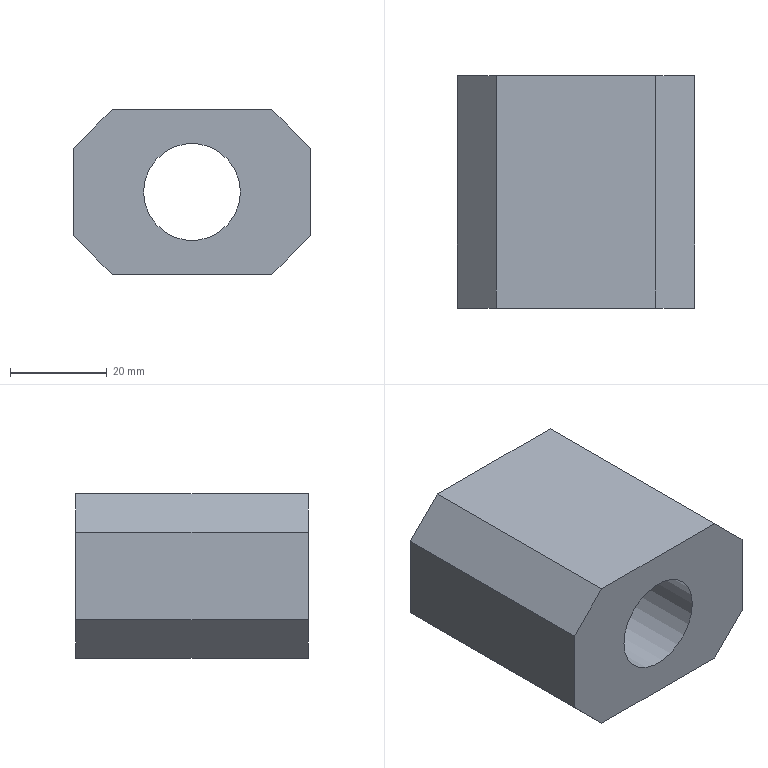Component | NX | NUT | 1 solid | 11 faces | box 49 x 48 x 34 mm | volume 58744 mm3 | plane 10 | cylinder 1 | commonest cylinder face diameters 20 x1
STEP:
#1=CARTESIAN_POINT('',(0.,0.,0.));
#2=DIRECTION('',(0.,0.,1.));
#3=DIRECTION('',(1.,0.,0.));
#4=AXIS2_PLACEMENT_3D('',#1,#2,#3);
#5=CARTESIAN_POINT('',(29.335,31.63,45.));
#6=VERTEX_POINT('',#5);
#7=CARTESIAN_POINT('',(29.335,31.63,63.));
#8=VERTEX_POINT('',#7);
#9=CARTESIAN_POINT('',(29.335,31.63,37.));
#10=DIRECTION('',(0.,0.,1.));
#11=VECTOR('',#10,1.);
#12=LINE('',#9,#11);
#13=CARTESIAN_POINT('',(29.335,-16.37,37.));
#14=DIRECTION('',(-1.,0.,0.));
#15=DIRECTION('',(0.,-1.,0.));
#16=AXIS2_PLACEMENT_3D('',#13,#14,#15);
#17=PLANE('',#16);
#18=CARTESIAN_POINT('',(-48.,0.));
#19=DIRECTION('',(0.,1.));
#20=VECTOR('',#19,1.);
#21=LINE('',#18,#20);
#22=(GEOMETRIC_REPRESENTATION_CONTEXT(2)PARAMETRIC_REPRESENTATION_CONTEXT()REPRESENTATION_CONTEXT('',''));
#23=DEFINITIONAL_REPRESENTATION('',(#21),#22);
#24=PCURVE('',#17,#23);
#25=CARTESIAN_POINT('',(4.835,31.63,54.));
#26=DIRECTION('',(0.,-1.,0.));
#27=DIRECTION('',(1.,0.,0.));
#28=AXIS2_PLACEMENT_3D('',#25,#26,#27);
#29=PLANE('',#28);
#30=CARTESIAN_POINT('',(24.5,-17.));
#31=DIRECTION('',(0.,1.));
#32=VECTOR('',#31,1.);
#33=LINE('',#30,#32);
#34=(GEOMETRIC_REPRESENTATION_CONTEXT(2)PARAMETRIC_REPRESENTATION_CONTEXT()REPRESENTATION_CONTEXT('',''));
#35=DEFINITIONAL_REPRESENTATION('',(#33),#34);
#36=PCURVE('',#29,#35);
#37=SURFACE_CURVE('',#12,(#24,#36),.PCURVE_S1.);
#38=EDGE_CURVE('',#6,#8,#37,.T.);
#39=ORIENTED_EDGE('',*,*,#38,.T.);
#40=CARTESIAN_POINT('',(29.335,-16.37,63.));
#41=VERTEX_POINT('',#40);
#42=CARTESIAN_POINT('',(29.335,-16.37,63.));
#43=DIRECTION('',(0.,-1.,0.));
#44=VECTOR('',#43,1.);
#45=LINE('',#42,#44);
#46=CARTESIAN_POINT('',(0.,26.));
#47=DIRECTION('',(1.,0.));
#48=VECTOR('',#47,1.);
#49=LINE('',#46,#48);
#50=(GEOMETRIC_REPRESENTATION_CONTEXT(2)PARAMETRIC_REPRESENTATION_CONTEXT()REPRESENTATION_CONTEXT('',''));
#51=DEFINITIONAL_REPRESENTATION('',(#49),#50);
#52=PCURVE('',#17,#51);
#53=CARTESIAN_POINT('',(21.335,-16.37,71.));
#54=DIRECTION('',(-0.7071,0.,-0.7071));
#55=DIRECTION('',(0.,1.,0.));
#56=AXIS2_PLACEMENT_3D('',#53,#54,#55);
#57=PLANE('',#56);
#58=CARTESIAN_POINT('',(0.,11.314));
#59=DIRECTION('',(-1.,0.));
#60=VECTOR('',#59,1.);
#61=LINE('',#58,#60);
#62=(GEOMETRIC_REPRESENTATION_CONTEXT(2)PARAMETRIC_REPRESENTATION_CONTEXT()REPRESENTATION_CONTEXT('',''));
#63=DEFINITIONAL_REPRESENTATION('',(#61),#62);
#64=PCURVE('',#57,#63);
#65=SURFACE_CURVE('',#45,(#52,#64),.PCURVE_S1.);
#66=EDGE_CURVE('',#8,#41,#65,.T.);
#67=ORIENTED_EDGE('',*,*,#66,.T.);
#68=CARTESIAN_POINT('',(29.335,-16.37,45.));
#69=VERTEX_POINT('',#68);
#70=CARTESIAN_POINT('',(29.335,-16.37,37.));
#71=DIRECTION('',(0.,0.,1.));
#72=VECTOR('',#71,1.);
#73=LINE('',#70,#72);
#74=CARTESIAN_POINT('',(0.,0.));
#75=DIRECTION('',(0.,1.));
#76=VECTOR('',#75,1.);
#77=LINE('',#74,#76);
#78=(GEOMETRIC_REPRESENTATION_CONTEXT(2)PARAMETRIC_REPRESENTATION_CONTEXT()REPRESENTATION_CONTEXT('',''));
#79=DEFINITIONAL_REPRESENTATION('',(#77),#78);
#80=PCURVE('',#17,#79);
#81=CARTESIAN_POINT('',(4.835,-16.37,54.));
#82=DIRECTION('',(0.,-1.,0.));
#83=DIRECTION('',(1.,0.,0.));
#84=AXIS2_PLACEMENT_3D('',#81,#82,#83);
#85=PLANE('',#84);
#86=CARTESIAN_POINT('',(24.5,-17.));
#87=DIRECTION('',(0.,1.));
#88=VECTOR('',#87,1.);
#89=LINE('',#86,#88);
#90=(GEOMETRIC_REPRESENTATION_CONTEXT(2)PARAMETRIC_REPRESENTATION_CONTEXT()REPRESENTATION_CONTEXT('',''));
#91=DEFINITIONAL_REPRESENTATION('',(#89),#90);
#92=PCURVE('',#85,#91);
#93=SURFACE_CURVE('',#73,(#80,#92),.PCURVE_S1.);
#94=EDGE_CURVE('',#69,#41,#93,.T.);
#95=ORIENTED_EDGE('',*,*,#94,.F.);
#96=CARTESIAN_POINT('',(29.335,-16.37,45.));
#97=DIRECTION('',(0.,1.,0.));
#98=VECTOR('',#97,1.);
#99=LINE('',#96,#98);
#100=CARTESIAN_POINT('',(0.,8.));
#101=DIRECTION('',(-1.,0.));
#102=VECTOR('',#101,1.);
#103=LINE('',#100,#102);
#104=(GEOMETRIC_REPRESENTATION_CONTEXT(2)PARAMETRIC_REPRESENTATION_CONTEXT()REPRESENTATION_CONTEXT('',''));
#105=DEFINITIONAL_REPRESENTATION('',(#103),#104);
#106=PCURVE('',#17,#105);
#107=CARTESIAN_POINT('',(29.335,-16.37,45.));
#108=DIRECTION('',(-0.7071,0.,0.7071));
#109=DIRECTION('',(0.,1.,0.));
#110=AXIS2_PLACEMENT_3D('',#107,#108,#109);
#111=PLANE('',#110);
#112=CARTESIAN_POINT('',(0.,0.));
#113=DIRECTION('',(1.,0.));
#114=VECTOR('',#113,1.);
#115=LINE('',#112,#114);
#116=(GEOMETRIC_REPRESENTATION_CONTEXT(2)PARAMETRIC_REPRESENTATION_CONTEXT()REPRESENTATION_CONTEXT('',''));
#117=DEFINITIONAL_REPRESENTATION('',(#115),#116);
#118=PCURVE('',#111,#117);
#119=SURFACE_CURVE('',#99,(#106,#118),.PCURVE_S1.);
#120=EDGE_CURVE('',#69,#6,#119,.T.);
#121=ORIENTED_EDGE('',*,*,#120,.T.);
#122=EDGE_LOOP('',(#39,#67,#95,#121));
#123=FACE_BOUND('',#122,.T.);
#124=ADVANCED_FACE('',(#123),#17,.F.);
#125=CARTESIAN_POINT('',(21.335,31.63,71.));
#126=VERTEX_POINT('',#125);
#127=CARTESIAN_POINT('',(-11.665,31.63,71.));
#128=VERTEX_POINT('',#127);
#129=CARTESIAN_POINT('',(29.335,31.63,71.));
#130=DIRECTION('',(-1.,0.,0.));
#131=VECTOR('',#130,1.);
#132=LINE('',#129,#131);
#133=CARTESIAN_POINT('',(29.335,-16.37,71.));
#134=DIRECTION('',(0.,0.,-1.));
#135=DIRECTION('',(0.,1.,0.));
#136=AXIS2_PLACEMENT_3D('',#133,#134,#135);
#137=PLANE('',#136);
#138=CARTESIAN_POINT('',(48.,0.));
#139=DIRECTION('',(0.,-1.));
#140=VECTOR('',#139,1.);
#141=LINE('',#138,#140);
#142=(GEOMETRIC_REPRESENTATION_CONTEXT(2)PARAMETRIC_REPRESENTATION_CONTEXT()REPRESENTATION_CONTEXT('',''));
#143=DEFINITIONAL_REPRESENTATION('',(#141),#142);
#144=PCURVE('',#137,#143);
#145=CARTESIAN_POINT('',(24.5,17.));
#146=DIRECTION('',(-1.,0.));
#147=VECTOR('',#146,1.);
#148=LINE('',#145,#147);
#149=(GEOMETRIC_REPRESENTATION_CONTEXT(2)PARAMETRIC_REPRESENTATION_CONTEXT()REPRESENTATION_CONTEXT('',''));
#150=DEFINITIONAL_REPRESENTATION('',(#148),#149);
#151=PCURVE('',#29,#150);
#152=SURFACE_CURVE('',#132,(#144,#151),.PCURVE_S1.);
#153=EDGE_CURVE('',#126,#128,#152,.T.);
#154=ORIENTED_EDGE('',*,*,#153,.T.);
#155=CARTESIAN_POINT('',(-11.665,-16.37,71.));
#156=VERTEX_POINT('',#155);
#157=CARTESIAN_POINT('',(-11.665,-16.37,71.));
#158=DIRECTION('',(0.,-1.,0.));
#159=VECTOR('',#158,1.);
#160=LINE('',#157,#159);
#161=CARTESIAN_POINT('',(0.,-41.));
#162=DIRECTION('',(-1.,0.));
#163=VECTOR('',#162,1.);
#164=LINE('',#161,#163);
#165=(GEOMETRIC_REPRESENTATION_CONTEXT(2)PARAMETRIC_REPRESENTATION_CONTEXT()REPRESENTATION_CONTEXT('',''));
#166=DEFINITIONAL_REPRESENTATION('',(#164),#165);
#167=PCURVE('',#137,#166);
#168=CARTESIAN_POINT('',(-19.665,-16.37,63.));
#169=DIRECTION('',(0.7071,0.,-0.7071));
#170=DIRECTION('',(0.,1.,0.));
#171=AXIS2_PLACEMENT_3D('',#168,#169,#170);
#172=PLANE('',#171);
#173=CARTESIAN_POINT('',(0.,11.314));
#174=DIRECTION('',(-1.,0.));
#175=VECTOR('',#174,1.);
#176=LINE('',#173,#175);
#177=(GEOMETRIC_REPRESENTATION_CONTEXT(2)PARAMETRIC_REPRESENTATION_CONTEXT()REPRESENTATION_CONTEXT('',''));
#178=DEFINITIONAL_REPRESENTATION('',(#176),#177);
#179=PCURVE('',#172,#178);
#180=SURFACE_CURVE('',#160,(#167,#179),.PCURVE_S1.);
#181=EDGE_CURVE('',#128,#156,#180,.T.);
#182=ORIENTED_EDGE('',*,*,#181,.T.);
#183=CARTESIAN_POINT('',(21.335,-16.37,71.));
#184=VERTEX_POINT('',#183);
#185=CARTESIAN_POINT('',(29.335,-16.37,71.));
#186=DIRECTION('',(-1.,0.,0.));
#187=VECTOR('',#186,1.);
#188=LINE('',#185,#187);
#189=CARTESIAN_POINT('',(0.,0.));
#190=DIRECTION('',(0.,-1.));
#191=VECTOR('',#190,1.);
#192=LINE('',#189,#191);
#193=(GEOMETRIC_REPRESENTATION_CONTEXT(2)PARAMETRIC_REPRESENTATION_CONTEXT()REPRESENTATION_CONTEXT('',''));
#194=DEFINITIONAL_REPRESENTATION('',(#192),#193);
#195=PCURVE('',#137,#194);
#196=CARTESIAN_POINT('',(24.5,17.));
#197=DIRECTION('',(-1.,0.));
#198=VECTOR('',#197,1.);
#199=LINE('',#196,#198);
#200=(GEOMETRIC_REPRESENTATION_CONTEXT(2)PARAMETRIC_REPRESENTATION_CONTEXT()REPRESENTATION_CONTEXT('',''));
#201=DEFINITIONAL_REPRESENTATION('',(#199),#200);
#202=PCURVE('',#85,#201);
#203=SURFACE_CURVE('',#188,(#195,#202),.PCURVE_S1.);
#204=EDGE_CURVE('',#184,#156,#203,.T.);
#205=ORIENTED_EDGE('',*,*,#204,.F.);
#206=CARTESIAN_POINT('',(21.335,-16.37,71.));
#207=DIRECTION('',(0.,1.,0.));
#208=VECTOR('',#207,1.);
#209=LINE('',#206,#208);
#210=CARTESIAN_POINT('',(0.,-8.));
#211=DIRECTION('',(1.,0.));
#212=VECTOR('',#211,1.);
#213=LINE('',#210,#212);
#214=(GEOMETRIC_REPRESENTATION_CONTEXT(2)PARAMETRIC_REPRESENTATION_CONTEXT()REPRESENTATION_CONTEXT('',''));
#215=DEFINITIONAL_REPRESENTATION('',(#213),#214);
#216=PCURVE('',#137,#215);
#217=CARTESIAN_POINT('',(0.,0.));
#218=DIRECTION('',(1.,0.));
#219=VECTOR('',#218,1.);
#220=LINE('',#217,#219);
#221=(GEOMETRIC_REPRESENTATION_CONTEXT(2)PARAMETRIC_REPRESENTATION_CONTEXT()REPRESENTATION_CONTEXT('',''));
#222=DEFINITIONAL_REPRESENTATION('',(#220),#221);
#223=PCURVE('',#57,#222);
#224=SURFACE_CURVE('',#209,(#216,#223),.PCURVE_S1.);
#225=EDGE_CURVE('',#184,#126,#224,.T.);
#226=ORIENTED_EDGE('',*,*,#225,.T.);
#227=EDGE_LOOP('',(#154,#182,#205,#226));
#228=FACE_BOUND('',#227,.T.);
#229=ADVANCED_FACE('',(#228),#137,.F.);
#230=CARTESIAN_POINT('',(-19.665,-16.37,63.));
#231=VERTEX_POINT('',#230);
#232=CARTESIAN_POINT('',(-19.665,-16.37,45.));
#233=VERTEX_POINT('',#232);
#234=CARTESIAN_POINT('',(-19.665,-16.37,71.));
#235=DIRECTION('',(0.,0.,-1.));
#236=VECTOR('',#235,1.);
#237=LINE('',#234,#236);
#238=CARTESIAN_POINT('',(-19.665,-16.37,71.));
#239=DIRECTION('',(1.,0.,0.));
#240=DIRECTION('',(0.,1.,0.));
#241=AXIS2_PLACEMENT_3D('',#238,#239,#240);
#242=PLANE('',#241);
#243=CARTESIAN_POINT('',(0.,0.));
#244=DIRECTION('',(0.,-1.));
#245=VECTOR('',#244,1.);
#246=LINE('',#243,#245);
#247=(GEOMETRIC_REPRESENTATION_CONTEXT(2)PARAMETRIC_REPRESENTATION_CONTEXT()REPRESENTATION_CONTEXT('',''));
#248=DEFINITIONAL_REPRESENTATION('',(#246),#247);
#249=PCURVE('',#242,#248);
#250=CARTESIAN_POINT('',(-24.5,17.));
#251=DIRECTION('',(0.,-1.));
#252=VECTOR('',#251,1.);
#253=LINE('',#250,#252);
#254=(GEOMETRIC_REPRESENTATION_CONTEXT(2)PARAMETRIC_REPRESENTATION_CONTEXT()REPRESENTATION_CONTEXT('',''));
#255=DEFINITIONAL_REPRESENTATION('',(#253),#254);
#256=PCURVE('',#85,#255);
#257=SURFACE_CURVE('',#237,(#249,#256),.PCURVE_S1.);
#258=EDGE_CURVE('',#231,#233,#257,.T.);
#259=ORIENTED_EDGE('',*,*,#258,.F.);
#260=CARTESIAN_POINT('',(-19.665,31.63,63.));
#261=VERTEX_POINT('',#260);
#262=CARTESIAN_POINT('',(-19.665,-16.37,63.));
#263=DIRECTION('',(0.,1.,0.));
#264=VECTOR('',#263,1.);
#265=LINE('',#262,#264);
#266=CARTESIAN_POINT('',(0.,-8.));
#267=DIRECTION('',(1.,0.));
#268=VECTOR('',#267,1.);
#269=LINE('',#266,#268);
#270=(GEOMETRIC_REPRESENTATION_CONTEXT(2)PARAMETRIC_REPRESENTATION_CONTEXT()REPRESENTATION_CONTEXT('',''));
#271=DEFINITIONAL_REPRESENTATION('',(#269),#270);
#272=PCURVE('',#242,#271);
#273=CARTESIAN_POINT('',(0.,0.));
#274=DIRECTION('',(1.,0.));
#275=VECTOR('',#274,1.);
#276=LINE('',#273,#275);
#277=(GEOMETRIC_REPRESENTATION_CONTEXT(2)PARAMETRIC_REPRESENTATION_CONTEXT()REPRESENTATION_CONTEXT('',''));
#278=DEFINITIONAL_REPRESENTATION('',(#276),#277);
#279=PCURVE('',#172,#278);
#280=SURFACE_CURVE('',#265,(#272,#279),.PCURVE_S1.);
#281=EDGE_CURVE('',#231,#261,#280,.T.);
#282=ORIENTED_EDGE('',*,*,#281,.T.);
#283=CARTESIAN_POINT('',(-19.665,31.63,45.));
#284=VERTEX_POINT('',#283);
#285=CARTESIAN_POINT('',(-19.665,31.63,71.));
#286=DIRECTION('',(0.,0.,-1.));
#287=VECTOR('',#286,1.);
#288=LINE('',#285,#287);
#289=CARTESIAN_POINT('',(48.,0.));
#290=DIRECTION('',(0.,-1.));
#291=VECTOR('',#290,1.);
#292=LINE('',#289,#291);
#293=(GEOMETRIC_REPRESENTATION_CONTEXT(2)PARAMETRIC_REPRESENTATION_CONTEXT()REPRESENTATION_CONTEXT('',''));
#294=DEFINITIONAL_REPRESENTATION('',(#292),#293);
#295=PCURVE('',#242,#294);
#296=CARTESIAN_POINT('',(-24.5,17.));
#297=DIRECTION('',(0.,-1.));
#298=VECTOR('',#297,1.);
#299=LINE('',#296,#298);
#300=(GEOMETRIC_REPRESENTATION_CONTEXT(2)PARAMETRIC_REPRESENTATION_CONTEXT()REPRESENTATION_CONTEXT('',''));
#301=DEFINITIONAL_REPRESENTATION('',(#299),#300);
#302=PCURVE('',#29,#301);
#303=SURFACE_CURVE('',#288,(#295,#302),.PCURVE_S1.);
#304=EDGE_CURVE('',#261,#284,#303,.T.);
#305=ORIENTED_EDGE('',*,*,#304,.T.);
#306=CARTESIAN_POINT('',(-19.665,-16.37,45.));
#307=DIRECTION('',(0.,-1.,0.));
#308=VECTOR('',#307,1.);
#309=LINE('',#306,#308);
#310=CARTESIAN_POINT('',(0.,-26.));
#311=DIRECTION('',(-1.,0.));
#312=VECTOR('',#311,1.);
#313=LINE('',#310,#312);
#314=(GEOMETRIC_REPRESENTATION_CONTEXT(2)PARAMETRIC_REPRESENTATION_CONTEXT()REPRESENTATION_CONTEXT('',''));
#315=DEFINITIONAL_REPRESENTATION('',(#313),#314);
#316=PCURVE('',#242,#315);
#317=CARTESIAN_POINT('',(-11.665,-16.37,37.));
#318=DIRECTION('',(0.7071,0.,0.7071));
#319=DIRECTION('',(0.,1.,0.));
#320=AXIS2_PLACEMENT_3D('',#317,#318,#319);
#321=PLANE('',#320);
#322=CARTESIAN_POINT('',(0.,11.314));
#323=DIRECTION('',(-1.,0.));
#324=VECTOR('',#323,1.);
#325=LINE('',#322,#324);
#326=(GEOMETRIC_REPRESENTATION_CONTEXT(2)PARAMETRIC_REPRESENTATION_CONTEXT()REPRESENTATION_CONTEXT('',''));
#327=DEFINITIONAL_REPRESENTATION('',(#325),#326);
#328=PCURVE('',#321,#327);
#329=SURFACE_CURVE('',#309,(#316,#328),.PCURVE_S1.);
#330=EDGE_CURVE('',#284,#233,#329,.T.);
#331=ORIENTED_EDGE('',*,*,#330,.T.);
#332=EDGE_LOOP('',(#259,#282,#305,#331));
#333=FACE_BOUND('',#332,.T.);
#334=ADVANCED_FACE('',(#333),#242,.F.);
#335=CARTESIAN_POINT('',(-11.665,-16.37,37.));
#336=VERTEX_POINT('',#335);
#337=CARTESIAN_POINT('',(21.335,-16.37,37.));
#338=VERTEX_POINT('',#337);
#339=CARTESIAN_POINT('',(-19.665,-16.37,37.));
#340=DIRECTION('',(1.,0.,0.));
#341=VECTOR('',#340,1.);
#342=LINE('',#339,#341);
#343=CARTESIAN_POINT('',(-19.665,-16.37,37.));
#344=DIRECTION('',(0.,0.,1.));
#345=DIRECTION('',(0.,-1.,0.));
#346=AXIS2_PLACEMENT_3D('',#343,#344,#345);
#347=PLANE('',#346);
#348=CARTESIAN_POINT('',(0.,0.));
#349=DIRECTION('',(0.,1.));
#350=VECTOR('',#349,1.);
#351=LINE('',#348,#350);
#352=(GEOMETRIC_REPRESENTATION_CONTEXT(2)PARAMETRIC_REPRESENTATION_CONTEXT()REPRESENTATION_CONTEXT('',''));
#353=DEFINITIONAL_REPRESENTATION('',(#351),#352);
#354=PCURVE('',#347,#353);
#355=CARTESIAN_POINT('',(-24.5,-17.));
#356=DIRECTION('',(1.,0.));
#357=VECTOR('',#356,1.);
#358=LINE('',#355,#357);
#359=(GEOMETRIC_REPRESENTATION_CONTEXT(2)PARAMETRIC_REPRESENTATION_CONTEXT()REPRESENTATION_CONTEXT('',''));
#360=DEFINITIONAL_REPRESENTATION('',(#358),#359);
#361=PCURVE('',#85,#360);
#362=SURFACE_CURVE('',#342,(#354,#361),.PCURVE_S1.);
#363=EDGE_CURVE('',#336,#338,#362,.T.);
#364=ORIENTED_EDGE('',*,*,#363,.F.);
#365=CARTESIAN_POINT('',(-11.665,31.63,37.));
#366=VERTEX_POINT('',#365);
#367=CARTESIAN_POINT('',(-11.665,-16.37,37.));
#368=DIRECTION('',(0.,1.,0.));
#369=VECTOR('',#368,1.);
#370=LINE('',#367,#369);
#371=CARTESIAN_POINT('',(0.,8.));
#372=DIRECTION('',(-1.,0.));
#373=VECTOR('',#372,1.);
#374=LINE('',#371,#373);
#375=(GEOMETRIC_REPRESENTATION_CONTEXT(2)PARAMETRIC_REPRESENTATION_CONTEXT()REPRESENTATION_CONTEXT('',''));
#376=DEFINITIONAL_REPRESENTATION('',(#374),#375);
#377=PCURVE('',#347,#376);
#378=CARTESIAN_POINT('',(0.,0.));
#379=DIRECTION('',(1.,0.));
#380=VECTOR('',#379,1.);
#381=LINE('',#378,#380);
#382=(GEOMETRIC_REPRESENTATION_CONTEXT(2)PARAMETRIC_REPRESENTATION_CONTEXT()REPRESENTATION_CONTEXT('',''));
#383=DEFINITIONAL_REPRESENTATION('',(#381),#382);
#384=PCURVE('',#321,#383);
#385=SURFACE_CURVE('',#370,(#377,#384),.PCURVE_S1.);
#386=EDGE_CURVE('',#336,#366,#385,.T.);
#387=ORIENTED_EDGE('',*,*,#386,.T.);
#388=CARTESIAN_POINT('',(21.335,31.63,37.));
#389=VERTEX_POINT('',#388);
#390=CARTESIAN_POINT('',(-19.665,31.63,37.));
#391=DIRECTION('',(1.,0.,0.));
#392=VECTOR('',#391,1.);
#393=LINE('',#390,#392);
#394=CARTESIAN_POINT('',(-48.,0.));
#395=DIRECTION('',(0.,1.));
#396=VECTOR('',#395,1.);
#397=LINE('',#394,#396);
#398=(GEOMETRIC_REPRESENTATION_CONTEXT(2)PARAMETRIC_REPRESENTATION_CONTEXT()REPRESENTATION_CONTEXT('',''));
#399=DEFINITIONAL_REPRESENTATION('',(#397),#398);
#400=PCURVE('',#347,#399);
#401=CARTESIAN_POINT('',(-24.5,-17.));
#402=DIRECTION('',(1.,0.));
#403=VECTOR('',#402,1.);
#404=LINE('',#401,#403);
#405=(GEOMETRIC_REPRESENTATION_CONTEXT(2)PARAMETRIC_REPRESENTATION_CONTEXT()REPRESENTATION_CONTEXT('',''));
#406=DEFINITIONAL_REPRESENTATION('',(#404),#405);
#407=PCURVE('',#29,#406);
#408=SURFACE_CURVE('',#393,(#400,#407),.PCURVE_S1.);
#409=EDGE_CURVE('',#366,#389,#408,.T.);
#410=ORIENTED_EDGE('',*,*,#409,.T.);
#411=CARTESIAN_POINT('',(21.335,-16.37,37.));
#412=DIRECTION('',(0.,-1.,0.));
#413=VECTOR('',#412,1.);
#414=LINE('',#411,#413);
#415=CARTESIAN_POINT('',(0.,41.));
#416=DIRECTION('',(1.,0.));
#417=VECTOR('',#416,1.);
#418=LINE('',#415,#417);
#419=(GEOMETRIC_REPRESENTATION_CONTEXT(2)PARAMETRIC_REPRESENTATION_CONTEXT()REPRESENTATION_CONTEXT('',''));
#420=DEFINITIONAL_REPRESENTATION('',(#418),#419);
#421=PCURVE('',#347,#420);
#422=CARTESIAN_POINT('',(0.,11.314));
#423=DIRECTION('',(-1.,0.));
#424=VECTOR('',#423,1.);
#425=LINE('',#422,#424);
#426=(GEOMETRIC_REPRESENTATION_CONTEXT(2)PARAMETRIC_REPRESENTATION_CONTEXT()REPRESENTATION_CONTEXT('',''));
#427=DEFINITIONAL_REPRESENTATION('',(#425),#426);
#428=PCURVE('',#111,#427);
#429=SURFACE_CURVE('',#414,(#421,#428),.PCURVE_S1.);
#430=EDGE_CURVE('',#389,#338,#429,.T.);
#431=ORIENTED_EDGE('',*,*,#430,.T.);
#432=EDGE_LOOP('',(#364,#387,#410,#431));
#433=FACE_BOUND('',#432,.T.);
#434=ADVANCED_FACE('',(#433),#347,.F.);
#435=CARTESIAN_POINT('',(14.835,-16.37,54.));
#436=VERTEX_POINT('',#435);
#437=CARTESIAN_POINT('',(4.835,-16.37,54.));
#438=DIRECTION('',(0.,-1.,0.));
#439=DIRECTION('',(1.,0.,0.));
#440=AXIS2_PLACEMENT_3D('',#437,#438,#439);
#441=CIRCLE('',#440,10.);
#442=CARTESIAN_POINT('',(0.,0.));
#443=DIRECTION('',(1.,0.));
#444=AXIS2_PLACEMENT_2D('',#442,#443);
#445=CIRCLE('',#444,10.);
#446=(GEOMETRIC_REPRESENTATION_CONTEXT(2)PARAMETRIC_REPRESENTATION_CONTEXT()REPRESENTATION_CONTEXT('',''));
#447=DEFINITIONAL_REPRESENTATION('',(#445),#446);
#448=PCURVE('',#85,#447);
#449=CARTESIAN_POINT('',(4.835,31.63,54.));
#450=DIRECTION('',(0.,-1.,0.));
#451=DIRECTION('',(1.,0.,0.));
#452=AXIS2_PLACEMENT_3D('',#449,#450,#451);
#453=CYLINDRICAL_SURFACE('',#452,10.);
#454=CARTESIAN_POINT('',(0.,48.));
#455=DIRECTION('',(1.,0.));
#456=VECTOR('',#455,1.);
#457=LINE('',#454,#456);
#458=(GEOMETRIC_REPRESENTATION_CONTEXT(2)PARAMETRIC_REPRESENTATION_CONTEXT()REPRESENTATION_CONTEXT('',''));
#459=DEFINITIONAL_REPRESENTATION('',(#457),#458);
#460=PCURVE('',#453,#459);
#461=SURFACE_CURVE('',#441,(#448,#460),.PCURVE_S1.);
#462=EDGE_CURVE('',#436,#436,#461,.T.);
#463=ORIENTED_EDGE('',*,*,#462,.F.);
#464=EDGE_LOOP('',(#463));
#465=FACE_BOUND('',#464,.T.);
#466=ORIENTED_EDGE('',*,*,#204,.T.);
#467=CARTESIAN_POINT('',(-11.915,-16.37,70.75));
#468=DIRECTION('',(-0.7071,0.,-0.7071));
#469=VECTOR('',#468,1.);
#470=LINE('',#467,#469);
#471=CARTESIAN_POINT('',(-16.75,16.75));
#472=DIRECTION('',(-0.7071,-0.7071));
#473=VECTOR('',#472,1.);
#474=LINE('',#471,#473);
#475=(GEOMETRIC_REPRESENTATION_CONTEXT(2)PARAMETRIC_REPRESENTATION_CONTEXT()REPRESENTATION_CONTEXT('',''));
#476=DEFINITIONAL_REPRESENTATION('',(#474),#475);
#477=PCURVE('',#85,#476);
#478=CARTESIAN_POINT('',(0.,10.96));
#479=DIRECTION('',(0.,-1.));
#480=VECTOR('',#479,1.);
#481=LINE('',#478,#480);
#482=(GEOMETRIC_REPRESENTATION_CONTEXT(2)PARAMETRIC_REPRESENTATION_CONTEXT()REPRESENTATION_CONTEXT('',''));
#483=DEFINITIONAL_REPRESENTATION('',(#481),#482);
#484=PCURVE('',#172,#483);
#485=SURFACE_CURVE('',#470,(#477,#484),.PCURVE_S1.);
#486=EDGE_CURVE('',#156,#231,#485,.T.);
#487=ORIENTED_EDGE('',*,*,#486,.T.);
#488=ORIENTED_EDGE('',*,*,#258,.T.);
#489=CARTESIAN_POINT('',(-11.915,-16.37,37.25));
#490=DIRECTION('',(0.7071,0.,-0.7071));
#491=VECTOR('',#490,1.);
#492=LINE('',#489,#491);
#493=CARTESIAN_POINT('',(-16.75,-16.75));
#494=DIRECTION('',(0.7071,-0.7071));
#495=VECTOR('',#494,1.);
#496=LINE('',#493,#495);
#497=(GEOMETRIC_REPRESENTATION_CONTEXT(2)PARAMETRIC_REPRESENTATION_CONTEXT()REPRESENTATION_CONTEXT('',''));
#498=DEFINITIONAL_REPRESENTATION('',(#496),#497);
#499=PCURVE('',#85,#498);
#500=CARTESIAN_POINT('',(0.,0.3536));
#501=DIRECTION('',(0.,-1.));
#502=VECTOR('',#501,1.);
#503=LINE('',#500,#502);
#504=(GEOMETRIC_REPRESENTATION_CONTEXT(2)PARAMETRIC_REPRESENTATION_CONTEXT()REPRESENTATION_CONTEXT('',''));
#505=DEFINITIONAL_REPRESENTATION('',(#503),#504);
#506=PCURVE('',#321,#505);
#507=SURFACE_CURVE('',#492,(#499,#506),.PCURVE_S1.);
#508=EDGE_CURVE('',#233,#336,#507,.T.);
#509=ORIENTED_EDGE('',*,*,#508,.T.);
#510=ORIENTED_EDGE('',*,*,#363,.T.);
#511=CARTESIAN_POINT('',(21.585,-16.37,37.25));
#512=DIRECTION('',(0.7071,0.,0.7071));
#513=VECTOR('',#512,1.);
#514=LINE('',#511,#513);
#515=CARTESIAN_POINT('',(16.75,-16.75));
#516=DIRECTION('',(0.7071,0.7071));
#517=VECTOR('',#516,1.);
#518=LINE('',#515,#517);
#519=(GEOMETRIC_REPRESENTATION_CONTEXT(2)PARAMETRIC_REPRESENTATION_CONTEXT()REPRESENTATION_CONTEXT('',''));
#520=DEFINITIONAL_REPRESENTATION('',(#518),#519);
#521=PCURVE('',#85,#520);
#522=CARTESIAN_POINT('',(0.,10.96));
#523=DIRECTION('',(0.,-1.));
#524=VECTOR('',#523,1.);
#525=LINE('',#522,#524);
#526=(GEOMETRIC_REPRESENTATION_CONTEXT(2)PARAMETRIC_REPRESENTATION_CONTEXT()REPRESENTATION_CONTEXT('',''));
#527=DEFINITIONAL_REPRESENTATION('',(#525),#526);
#528=PCURVE('',#111,#527);
#529=SURFACE_CURVE('',#514,(#521,#528),.PCURVE_S1.);
#530=EDGE_CURVE('',#338,#69,#529,.T.);
#531=ORIENTED_EDGE('',*,*,#530,.T.);
#532=ORIENTED_EDGE('',*,*,#94,.T.);
#533=CARTESIAN_POINT('',(21.585,-16.37,70.75));
#534=DIRECTION('',(-0.7071,0.,0.7071));
#535=VECTOR('',#534,1.);
#536=LINE('',#533,#535);
#537=CARTESIAN_POINT('',(16.75,16.75));
#538=DIRECTION('',(-0.7071,0.7071));
#539=VECTOR('',#538,1.);
#540=LINE('',#537,#539);
#541=(GEOMETRIC_REPRESENTATION_CONTEXT(2)PARAMETRIC_REPRESENTATION_CONTEXT()REPRESENTATION_CONTEXT('',''));
#542=DEFINITIONAL_REPRESENTATION('',(#540),#541);
#543=PCURVE('',#85,#542);
#544=CARTESIAN_POINT('',(0.,0.3536));
#545=DIRECTION('',(0.,-1.));
#546=VECTOR('',#545,1.);
#547=LINE('',#544,#546);
#548=(GEOMETRIC_REPRESENTATION_CONTEXT(2)PARAMETRIC_REPRESENTATION_CONTEXT()REPRESENTATION_CONTEXT('',''));
#549=DEFINITIONAL_REPRESENTATION('',(#547),#548);
#550=PCURVE('',#57,#549);
#551=SURFACE_CURVE('',#536,(#543,#550),.PCURVE_S1.);
#552=EDGE_CURVE('',#41,#184,#551,.T.);
#553=ORIENTED_EDGE('',*,*,#552,.T.);
#554=EDGE_LOOP('',(#466,#487,#488,#509,#510,#531,#532,#553));
#555=FACE_BOUND('',#554,.T.);
#556=ADVANCED_FACE('',(#465,#555),#85,.T.);
#557=CARTESIAN_POINT('',(14.835,31.63,54.));
#558=VERTEX_POINT('',#557);
#559=CARTESIAN_POINT('',(4.835,31.63,54.));
#560=DIRECTION('',(0.,-1.,0.));
#561=DIRECTION('',(1.,0.,0.));
#562=AXIS2_PLACEMENT_3D('',#559,#560,#561);
#563=CIRCLE('',#562,10.);
#564=CARTESIAN_POINT('',(0.,0.));
#565=DIRECTION('',(1.,0.));
#566=AXIS2_PLACEMENT_2D('',#564,#565);
#567=CIRCLE('',#566,10.);
#568=(GEOMETRIC_REPRESENTATION_CONTEXT(2)PARAMETRIC_REPRESENTATION_CONTEXT()REPRESENTATION_CONTEXT('',''));
#569=DEFINITIONAL_REPRESENTATION('',(#567),#568);
#570=PCURVE('',#29,#569);
#571=CARTESIAN_POINT('',(0.,0.));
#572=DIRECTION('',(1.,0.));
#573=VECTOR('',#572,1.);
#574=LINE('',#571,#573);
#575=(GEOMETRIC_REPRESENTATION_CONTEXT(2)PARAMETRIC_REPRESENTATION_CONTEXT()REPRESENTATION_CONTEXT('',''));
#576=DEFINITIONAL_REPRESENTATION('',(#574),#575);
#577=PCURVE('',#453,#576);
#578=SURFACE_CURVE('',#563,(#570,#577),.PCURVE_S1.);
#579=EDGE_CURVE('',#558,#558,#578,.T.);
#580=ORIENTED_EDGE('',*,*,#579,.T.);
#581=EDGE_LOOP('',(#580));
#582=FACE_BOUND('',#581,.T.);
#583=ORIENTED_EDGE('',*,*,#304,.F.);
#584=CARTESIAN_POINT('',(-19.665,31.63,63.));
#585=DIRECTION('',(0.7071,0.,0.7071));
#586=VECTOR('',#585,1.);
#587=LINE('',#584,#586);
#588=CARTESIAN_POINT('',(-24.5,9.));
#589=DIRECTION('',(0.7071,0.7071));
#590=VECTOR('',#589,1.);
#591=LINE('',#588,#590);
#592=(GEOMETRIC_REPRESENTATION_CONTEXT(2)PARAMETRIC_REPRESENTATION_CONTEXT()REPRESENTATION_CONTEXT('',''));
#593=DEFINITIONAL_REPRESENTATION('',(#591),#592);
#594=PCURVE('',#29,#593);
#595=CARTESIAN_POINT('',(48.,0.));
#596=DIRECTION('',(0.,1.));
#597=VECTOR('',#596,1.);
#598=LINE('',#595,#597);
#599=(GEOMETRIC_REPRESENTATION_CONTEXT(2)PARAMETRIC_REPRESENTATION_CONTEXT()REPRESENTATION_CONTEXT('',''));
#600=DEFINITIONAL_REPRESENTATION('',(#598),#599);
#601=PCURVE('',#172,#600);
#602=SURFACE_CURVE('',#587,(#594,#601),.PCURVE_S1.);
#603=EDGE_CURVE('',#261,#128,#602,.T.);
#604=ORIENTED_EDGE('',*,*,#603,.T.);
#605=ORIENTED_EDGE('',*,*,#153,.F.);
#606=CARTESIAN_POINT('',(21.335,31.63,71.));
#607=DIRECTION('',(0.7071,0.,-0.7071));
#608=VECTOR('',#607,1.);
#609=LINE('',#606,#608);
#610=CARTESIAN_POINT('',(16.5,17.));
#611=DIRECTION('',(0.7071,-0.7071));
#612=VECTOR('',#611,1.);
#613=LINE('',#610,#612);
#614=(GEOMETRIC_REPRESENTATION_CONTEXT(2)PARAMETRIC_REPRESENTATION_CONTEXT()REPRESENTATION_CONTEXT('',''));
#615=DEFINITIONAL_REPRESENTATION('',(#613),#614);
#616=PCURVE('',#29,#615);
#617=CARTESIAN_POINT('',(48.,0.));
#618=DIRECTION('',(0.,1.));
#619=VECTOR('',#618,1.);
#620=LINE('',#617,#619);
#621=(GEOMETRIC_REPRESENTATION_CONTEXT(2)PARAMETRIC_REPRESENTATION_CONTEXT()REPRESENTATION_CONTEXT('',''));
#622=DEFINITIONAL_REPRESENTATION('',(#620),#621);
#623=PCURVE('',#57,#622);
#624=SURFACE_CURVE('',#609,(#616,#623),.PCURVE_S1.);
#625=EDGE_CURVE('',#126,#8,#624,.T.);
#626=ORIENTED_EDGE('',*,*,#625,.T.);
#627=ORIENTED_EDGE('',*,*,#38,.F.);
#628=CARTESIAN_POINT('',(29.335,31.63,45.));
#629=DIRECTION('',(-0.7071,0.,-0.7071));
#630=VECTOR('',#629,1.);
#631=LINE('',#628,#630);
#632=CARTESIAN_POINT('',(24.5,-9.));
#633=DIRECTION('',(-0.7071,-0.7071));
#634=VECTOR('',#633,1.);
#635=LINE('',#632,#634);
#636=(GEOMETRIC_REPRESENTATION_CONTEXT(2)PARAMETRIC_REPRESENTATION_CONTEXT()REPRESENTATION_CONTEXT('',''));
#637=DEFINITIONAL_REPRESENTATION('',(#635),#636);
#638=PCURVE('',#29,#637);
#639=CARTESIAN_POINT('',(48.,0.));
#640=DIRECTION('',(0.,1.));
#641=VECTOR('',#640,1.);
#642=LINE('',#639,#641);
#643=(GEOMETRIC_REPRESENTATION_CONTEXT(2)PARAMETRIC_REPRESENTATION_CONTEXT()REPRESENTATION_CONTEXT('',''));
#644=DEFINITIONAL_REPRESENTATION('',(#642),#643);
#645=PCURVE('',#111,#644);
#646=SURFACE_CURVE('',#631,(#638,#645),.PCURVE_S1.);
#647=EDGE_CURVE('',#6,#389,#646,.T.);
#648=ORIENTED_EDGE('',*,*,#647,.T.);
#649=ORIENTED_EDGE('',*,*,#409,.F.);
#650=CARTESIAN_POINT('',(-11.665,31.63,37.));
#651=DIRECTION('',(-0.7071,0.,0.7071));
#652=VECTOR('',#651,1.);
#653=LINE('',#650,#652);
#654=CARTESIAN_POINT('',(-16.5,-17.));
#655=DIRECTION('',(-0.7071,0.7071));
#656=VECTOR('',#655,1.);
#657=LINE('',#654,#656);
#658=(GEOMETRIC_REPRESENTATION_CONTEXT(2)PARAMETRIC_REPRESENTATION_CONTEXT()REPRESENTATION_CONTEXT('',''));
#659=DEFINITIONAL_REPRESENTATION('',(#657),#658);
#660=PCURVE('',#29,#659);
#661=CARTESIAN_POINT('',(48.,0.));
#662=DIRECTION('',(0.,1.));
#663=VECTOR('',#662,1.);
#664=LINE('',#661,#663);
#665=(GEOMETRIC_REPRESENTATION_CONTEXT(2)PARAMETRIC_REPRESENTATION_CONTEXT()REPRESENTATION_CONTEXT('',''));
#666=DEFINITIONAL_REPRESENTATION('',(#664),#665);
#667=PCURVE('',#321,#666);
#668=SURFACE_CURVE('',#653,(#660,#667),.PCURVE_S1.);
#669=EDGE_CURVE('',#366,#284,#668,.T.);
#670=ORIENTED_EDGE('',*,*,#669,.T.);
#671=EDGE_LOOP('',(#583,#604,#605,#626,#627,#648,#649,#670));
#672=FACE_BOUND('',#671,.T.);
#673=ADVANCED_FACE('',(#582,#672),#29,.F.);
#674=ORIENTED_EDGE('',*,*,#486,.F.);
#675=ORIENTED_EDGE('',*,*,#181,.F.);
#676=ORIENTED_EDGE('',*,*,#603,.F.);
#677=ORIENTED_EDGE('',*,*,#281,.F.);
#678=EDGE_LOOP('',(#674,#675,#676,#677));
#679=FACE_BOUND('',#678,.T.);
#680=ADVANCED_FACE('',(#679),#172,.F.);
#681=ORIENTED_EDGE('',*,*,#508,.F.);
#682=ORIENTED_EDGE('',*,*,#330,.F.);
#683=ORIENTED_EDGE('',*,*,#669,.F.);
#684=ORIENTED_EDGE('',*,*,#386,.F.);
#685=EDGE_LOOP('',(#681,#682,#683,#684));
#686=FACE_BOUND('',#685,.T.);
#687=ADVANCED_FACE('',(#686),#321,.F.);
#688=ORIENTED_EDGE('',*,*,#552,.F.);
#689=ORIENTED_EDGE('',*,*,#66,.F.);
#690=ORIENTED_EDGE('',*,*,#625,.F.);
#691=ORIENTED_EDGE('',*,*,#225,.F.);
#692=EDGE_LOOP('',(#688,#689,#690,#691));
#693=FACE_BOUND('',#692,.T.);
#694=ADVANCED_FACE('',(#693),#57,.F.);
#695=ORIENTED_EDGE('',*,*,#530,.F.);
#696=ORIENTED_EDGE('',*,*,#430,.F.);
#697=ORIENTED_EDGE('',*,*,#647,.F.);
#698=ORIENTED_EDGE('',*,*,#120,.F.);
#699=EDGE_LOOP('',(#695,#696,#697,#698));
#700=FACE_BOUND('',#699,.T.);
#701=ADVANCED_FACE('',(#700),#111,.F.);
#702=ORIENTED_EDGE('',*,*,#462,.F.);
#703=CARTESIAN_POINT('',(14.835,31.63,54.));
#704=CARTESIAN_POINT('',(14.835,-16.37,54.));
#705=B_SPLINE_CURVE_WITH_KNOTS('',1,(#703,#704),.UNSPECIFIED.,.F.,.F.,(2,2),(0.,48.),.PIECEWISE_BEZIER_KNOTS.);
#706=CARTESIAN_POINT('',(0.,0.));
#707=DIRECTION('',(0.,1.));
#708=VECTOR('',#707,1.);
#709=LINE('',#706,#708);
#710=(GEOMETRIC_REPRESENTATION_CONTEXT(2)PARAMETRIC_REPRESENTATION_CONTEXT()REPRESENTATION_CONTEXT('',''));
#711=DEFINITIONAL_REPRESENTATION('',(#709),#710);
#712=PCURVE('',#453,#711);
#713=CARTESIAN_POINT('',(6.283,0.));
#714=DIRECTION('',(0.,1.));
#715=VECTOR('',#714,1.);
#716=LINE('',#713,#715);
#717=(GEOMETRIC_REPRESENTATION_CONTEXT(2)PARAMETRIC_REPRESENTATION_CONTEXT()REPRESENTATION_CONTEXT('',''));
#718=DEFINITIONAL_REPRESENTATION('',(#716),#717);
#719=PCURVE('',#453,#718);
#720=SEAM_CURVE('',#705,(#712,#719),.PCURVE_S1.);
#721=EDGE_CURVE('',#558,#436,#720,.T.);
#722=ORIENTED_EDGE('',*,*,#721,.F.);
#723=ORIENTED_EDGE('',*,*,#579,.T.);
#724=ORIENTED_EDGE('',*,*,#721,.T.);
#725=EDGE_LOOP('',(#702,#722,#723,#724));
#726=FACE_BOUND('',#725,.F.);
#727=ADVANCED_FACE('',(#726),#453,.F.);
#728=CLOSED_SHELL('',(#124,#229,#334,#434,#556,#673,#680,#687,#694,#701,#727));
#729=MANIFOLD_SOLID_BREP('',#728);
#730=(LENGTH_UNIT()NAMED_UNIT(*)SI_UNIT(.MILLI.,.METRE.));
#731=UNCERTAINTY_MEASURE_WITH_UNIT(LENGTH_MEASURE(0.000001),#730,'','');
#732=(NAMED_UNIT(*)PLANE_ANGLE_UNIT()SI_UNIT($,.RADIAN.));
#733=(NAMED_UNIT(*)SI_UNIT($,.STERADIAN.)SOLID_ANGLE_UNIT());
#734=(GEOMETRIC_REPRESENTATION_CONTEXT(3)GLOBAL_UNCERTAINTY_ASSIGNED_CONTEXT((#731))GLOBAL_UNIT_ASSIGNED_CONTEXT((#730,#732,#733))REPRESENTATION_CONTEXT('',''));
#735=ADVANCED_BREP_SHAPE_REPRESENTATION('',(#4,#729),#734);